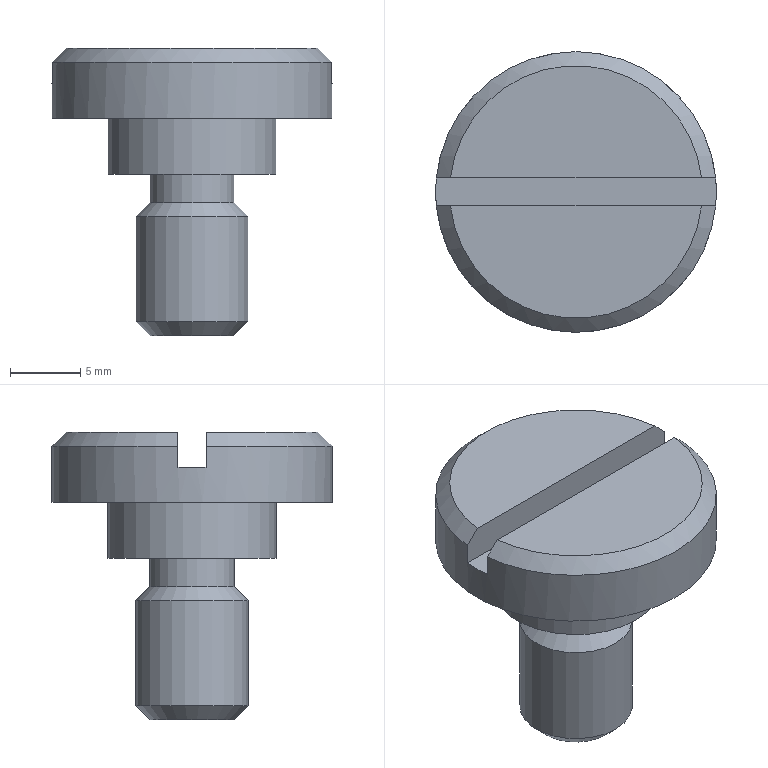Component | NX | DRILL_BUSHING_SCREW | 1 solid | 16 faces | box 20 x 20 x 20.5 mm | volume 2406 mm3 | plane 8 | cylinder 4 | cone 4 | commonest cylinder face diameters 8 x1 6 x1 12 x1 20 x1
STEP:
#1=CARTESIAN_POINT('',(0.,0.,0.));
#2=DIRECTION('',(0.,0.,1.));
#3=DIRECTION('',(1.,0.,0.));
#4=AXIS2_PLACEMENT_3D('',#1,#2,#3);
#5=CARTESIAN_POINT('',(-8.944,49.,-79.));
#6=VERTEX_POINT('',#5);
#7=CARTESIAN_POINT('',(8.944,49.,-79.));
#8=VERTEX_POINT('',#7);
#9=CARTESIAN_POINT('',(-13.1,49.,-79.));
#10=DIRECTION('',(1.,-0.,0.));
#11=VECTOR('',#10,1.);
#12=LINE('',#9,#11);
#13=CARTESIAN_POINT('',(-0.,50.,-79.));
#14=DIRECTION('',(0.,0.,1.));
#15=DIRECTION('',(0.,1.,0.));
#16=AXIS2_PLACEMENT_3D('',#13,#14,#15);
#17=PLANE('',#16);
#18=CARTESIAN_POINT('',(-1.,13.1));
#19=DIRECTION('',(-0.,-1.));
#20=VECTOR('',#19,1.);
#21=LINE('',#18,#20);
#22=(GEOMETRIC_REPRESENTATION_CONTEXT(2)PARAMETRIC_REPRESENTATION_CONTEXT()REPRESENTATION_CONTEXT('',''));
#23=DEFINITIONAL_REPRESENTATION('',(#21),#22);
#24=PCURVE('',#17,#23);
#25=CARTESIAN_POINT('',(-13.1,49.,-81.5));
#26=DIRECTION('',(-0.,-1.,0.));
#27=DIRECTION('',(1.,-0.,0.));
#28=AXIS2_PLACEMENT_3D('',#25,#26,#27);
#29=PLANE('',#28);
#30=CARTESIAN_POINT('',(0.,2.5));
#31=DIRECTION('',(1.,0.));
#32=VECTOR('',#31,1.);
#33=LINE('',#30,#32);
#34=(GEOMETRIC_REPRESENTATION_CONTEXT(2)PARAMETRIC_REPRESENTATION_CONTEXT()REPRESENTATION_CONTEXT('',''));
#35=DEFINITIONAL_REPRESENTATION('',(#33),#34);
#36=PCURVE('',#29,#35);
#37=SURFACE_CURVE('',#12,(#24,#36),.PCURVE_S1.);
#38=EDGE_CURVE('',#6,#8,#37,.T.);
#39=ORIENTED_EDGE('',*,*,#38,.F.);
#40=CARTESIAN_POINT('',(-0.,50.,-79.));
#41=DIRECTION('',(0.,0.,1.));
#42=DIRECTION('',(0.,1.,0.));
#43=AXIS2_PLACEMENT_3D('',#40,#41,#42);
#44=CIRCLE('',#43,9.);
#45=CARTESIAN_POINT('',(0.,0.));
#46=DIRECTION('',(1.,0.));
#47=AXIS2_PLACEMENT_2D('',#45,#46);
#48=CIRCLE('',#47,9.);
#49=(GEOMETRIC_REPRESENTATION_CONTEXT(2)PARAMETRIC_REPRESENTATION_CONTEXT()REPRESENTATION_CONTEXT('',''));
#50=DEFINITIONAL_REPRESENTATION('',(#48),#49);
#51=PCURVE('',#17,#50);
#52=CARTESIAN_POINT('',(-0.,50.,-79.));
#53=DIRECTION('',(0.,0.,-1.));
#54=DIRECTION('',(0.,-1.,0.));
#55=AXIS2_PLACEMENT_3D('',#52,#53,#54);
#56=CONICAL_SURFACE('',#55,9.,0.7854);
#57=CARTESIAN_POINT('',(3.142,0.));
#58=DIRECTION('',(-1.,0.));
#59=VECTOR('',#58,1.);
#60=LINE('',#57,#59);
#61=(GEOMETRIC_REPRESENTATION_CONTEXT(2)PARAMETRIC_REPRESENTATION_CONTEXT()REPRESENTATION_CONTEXT('',''));
#62=DEFINITIONAL_REPRESENTATION('',(#60),#61);
#63=PCURVE('',#56,#62);
#64=SURFACE_CURVE('',#44,(#51,#63),.PCURVE_S1.);
#65=EDGE_CURVE('',#6,#8,#64,.T.);
#66=ORIENTED_EDGE('',*,*,#65,.T.);
#67=EDGE_LOOP('',(#39,#66));
#68=FACE_BOUND('',#67,.T.);
#69=ADVANCED_FACE('',(#68),#17,.T.);
#70=CARTESIAN_POINT('',(-0.,54.,-98.5));
#71=VERTEX_POINT('',#70);
#72=CARTESIAN_POINT('',(-0.,50.,-98.5));
#73=DIRECTION('',(0.,0.,1.));
#74=DIRECTION('',(0.,1.,0.));
#75=AXIS2_PLACEMENT_3D('',#72,#73,#74);
#76=CIRCLE('',#75,4.);
#77=CARTESIAN_POINT('',(-0.,50.,-90.));
#78=DIRECTION('',(0.,0.,-1.));
#79=DIRECTION('',(0.,-1.,0.));
#80=AXIS2_PLACEMENT_3D('',#77,#78,#79);
#81=CYLINDRICAL_SURFACE('',#80,4.);
#82=CARTESIAN_POINT('',(9.425,8.5));
#83=DIRECTION('',(-1.,0.));
#84=VECTOR('',#83,1.);
#85=LINE('',#82,#84);
#86=(GEOMETRIC_REPRESENTATION_CONTEXT(2)PARAMETRIC_REPRESENTATION_CONTEXT()REPRESENTATION_CONTEXT('',''));
#87=DEFINITIONAL_REPRESENTATION('',(#85),#86);
#88=PCURVE('',#81,#87);
#89=CARTESIAN_POINT('',(-0.,50.,-98.5));
#90=DIRECTION('',(0.,0.,1.));
#91=DIRECTION('',(0.,1.,0.));
#92=AXIS2_PLACEMENT_3D('',#89,#90,#91);
#93=CONICAL_SURFACE('',#92,4.,0.7854);
#94=CARTESIAN_POINT('',(0.,0.));
#95=DIRECTION('',(1.,0.));
#96=VECTOR('',#95,1.);
#97=LINE('',#94,#96);
#98=(GEOMETRIC_REPRESENTATION_CONTEXT(2)PARAMETRIC_REPRESENTATION_CONTEXT()REPRESENTATION_CONTEXT('',''));
#99=DEFINITIONAL_REPRESENTATION('',(#97),#98);
#100=PCURVE('',#93,#99);
#101=SURFACE_CURVE('',#76,(#88,#100),.PCURVE_S1.);
#102=EDGE_CURVE('',#71,#71,#101,.T.);
#103=ORIENTED_EDGE('',*,*,#102,.T.);
#104=CARTESIAN_POINT('',(-0.,54.,-91.));
#105=VERTEX_POINT('',#104);
#106=CARTESIAN_POINT('',(-0.,54.,-91.));
#107=CARTESIAN_POINT('',(-0.,54.,-98.5));
#108=B_SPLINE_CURVE_WITH_KNOTS('',1,(#106,#107),.UNSPECIFIED.,.F.,.F.,(2,2),(1.,8.5),.PIECEWISE_BEZIER_KNOTS.);
#109=CARTESIAN_POINT('',(3.142,0.));
#110=DIRECTION('',(0.,1.));
#111=VECTOR('',#110,1.);
#112=LINE('',#109,#111);
#113=(GEOMETRIC_REPRESENTATION_CONTEXT(2)PARAMETRIC_REPRESENTATION_CONTEXT()REPRESENTATION_CONTEXT('',''));
#114=DEFINITIONAL_REPRESENTATION('',(#112),#113);
#115=PCURVE('',#81,#114);
#116=CARTESIAN_POINT('',(9.425,0.));
#117=DIRECTION('',(0.,1.));
#118=VECTOR('',#117,1.);
#119=LINE('',#116,#118);
#120=(GEOMETRIC_REPRESENTATION_CONTEXT(2)PARAMETRIC_REPRESENTATION_CONTEXT()REPRESENTATION_CONTEXT('',''));
#121=DEFINITIONAL_REPRESENTATION('',(#119),#120);
#122=PCURVE('',#81,#121);
#123=SEAM_CURVE('',#108,(#115,#122),.PCURVE_S1.);
#124=EDGE_CURVE('',#105,#71,#123,.T.);
#125=ORIENTED_EDGE('',*,*,#124,.F.);
#126=CARTESIAN_POINT('',(-0.,50.,-91.));
#127=DIRECTION('',(0.,0.,-1.));
#128=DIRECTION('',(0.,1.,0.));
#129=AXIS2_PLACEMENT_3D('',#126,#127,#128);
#130=CIRCLE('',#129,4.);
#131=CARTESIAN_POINT('',(3.142,1.));
#132=DIRECTION('',(1.,0.));
#133=VECTOR('',#132,1.);
#134=LINE('',#131,#133);
#135=(GEOMETRIC_REPRESENTATION_CONTEXT(2)PARAMETRIC_REPRESENTATION_CONTEXT()REPRESENTATION_CONTEXT('',''));
#136=DEFINITIONAL_REPRESENTATION('',(#134),#135);
#137=PCURVE('',#81,#136);
#138=CARTESIAN_POINT('',(-0.,50.,-90.));
#139=DIRECTION('',(0.,0.,-1.));
#140=DIRECTION('',(0.,-1.,0.));
#141=AXIS2_PLACEMENT_3D('',#138,#139,#140);
#142=CONICAL_SURFACE('',#141,3.,0.7854);
#143=CARTESIAN_POINT('',(3.142,1.));
#144=DIRECTION('',(1.,0.));
#145=VECTOR('',#144,1.);
#146=LINE('',#143,#145);
#147=(GEOMETRIC_REPRESENTATION_CONTEXT(2)PARAMETRIC_REPRESENTATION_CONTEXT()REPRESENTATION_CONTEXT('',''));
#148=DEFINITIONAL_REPRESENTATION('',(#146),#147);
#149=PCURVE('',#142,#148);
#150=SURFACE_CURVE('',#130,(#137,#149),.PCURVE_S1.);
#151=EDGE_CURVE('',#105,#105,#150,.T.);
#152=ORIENTED_EDGE('',*,*,#151,.T.);
#153=ORIENTED_EDGE('',*,*,#124,.T.);
#154=EDGE_LOOP('',(#103,#125,#152,#153));
#155=FACE_BOUND('',#154,.T.);
#156=ADVANCED_FACE('',(#155),#81,.T.);
#157=CARTESIAN_POINT('',(-0.,53.,-99.5));
#158=VERTEX_POINT('',#157);
#159=CARTESIAN_POINT('',(-0.,50.,-99.5));
#160=DIRECTION('',(0.,0.,-1.));
#161=DIRECTION('',(0.,1.,0.));
#162=AXIS2_PLACEMENT_3D('',#159,#160,#161);
#163=CIRCLE('',#162,3.);
#164=CARTESIAN_POINT('',(-0.,50.,-99.5));
#165=DIRECTION('',(0.,0.,1.));
#166=DIRECTION('',(0.,1.,0.));
#167=AXIS2_PLACEMENT_3D('',#164,#165,#166);
#168=PLANE('',#167);
#169=CARTESIAN_POINT('',(3.,0.));
#170=CARTESIAN_POINT('',(3.,-5.196));
#171=CARTESIAN_POINT('',(-1.5,-2.598));
#172=CARTESIAN_POINT('',(-6.,-0.));
#173=CARTESIAN_POINT('',(-1.5,2.598));
#174=CARTESIAN_POINT('',(3.,5.196));
#175=CARTESIAN_POINT('',(3.,0.));
#176=(BOUNDED_CURVE()B_SPLINE_CURVE(2,(#169,#170,#171,#172,#173,#174,#175),.UNSPECIFIED.,.T.,.F.)B_SPLINE_CURVE_WITH_KNOTS((1,2,2,2,2,1),(-2.094,0.,2.094,4.189,6.283,8.378),.UNSPECIFIED.)CURVE()GEOMETRIC_REPRESENTATION_ITEM()RATIONAL_B_SPLINE_CURVE((1.,0.5,1.,0.5,1.,0.5,1.))REPRESENTATION_ITEM(''));
#177=(GEOMETRIC_REPRESENTATION_CONTEXT(2)PARAMETRIC_REPRESENTATION_CONTEXT()REPRESENTATION_CONTEXT('',''));
#178=DEFINITIONAL_REPRESENTATION('',(#176),#177);
#179=PCURVE('',#168,#178);
#180=CARTESIAN_POINT('',(6.283,-1.));
#181=DIRECTION('',(-1.,0.));
#182=VECTOR('',#181,1.);
#183=LINE('',#180,#182);
#184=(GEOMETRIC_REPRESENTATION_CONTEXT(2)PARAMETRIC_REPRESENTATION_CONTEXT()REPRESENTATION_CONTEXT('',''));
#185=DEFINITIONAL_REPRESENTATION('',(#183),#184);
#186=PCURVE('',#93,#185);
#187=SURFACE_CURVE('',#163,(#179,#186),.PCURVE_S1.);
#188=EDGE_CURVE('',#158,#158,#187,.T.);
#189=ORIENTED_EDGE('',*,*,#188,.T.);
#190=EDGE_LOOP('',(#189));
#191=FACE_BOUND('',#190,.T.);
#192=ADVANCED_FACE('',(#191),#168,.F.);
#193=CARTESIAN_POINT('',(-0.,53.,-88.));
#194=VERTEX_POINT('',#193);
#195=CARTESIAN_POINT('',(-0.,50.,-88.));
#196=DIRECTION('',(0.,0.,1.));
#197=DIRECTION('',(0.,1.,0.));
#198=AXIS2_PLACEMENT_3D('',#195,#196,#197);
#199=CIRCLE('',#198,3.);
#200=CARTESIAN_POINT('',(-0.,50.,-88.));
#201=DIRECTION('',(0.,0.,-1.));
#202=DIRECTION('',(0.,-1.,0.));
#203=AXIS2_PLACEMENT_3D('',#200,#201,#202);
#204=CYLINDRICAL_SURFACE('',#203,3.);
#205=CARTESIAN_POINT('',(9.425,0.));
#206=DIRECTION('',(-1.,0.));
#207=VECTOR('',#206,1.);
#208=LINE('',#205,#207);
#209=(GEOMETRIC_REPRESENTATION_CONTEXT(2)PARAMETRIC_REPRESENTATION_CONTEXT()REPRESENTATION_CONTEXT('',''));
#210=DEFINITIONAL_REPRESENTATION('',(#208),#209);
#211=PCURVE('',#204,#210);
#212=CARTESIAN_POINT('',(-0.,50.,-88.));
#213=DIRECTION('',(0.,0.,1.));
#214=DIRECTION('',(0.,1.,0.));
#215=AXIS2_PLACEMENT_3D('',#212,#213,#214);
#216=PLANE('',#215);
#217=CARTESIAN_POINT('',(0.,0.));
#218=DIRECTION('',(1.,0.));
#219=AXIS2_PLACEMENT_2D('',#217,#218);
#220=CIRCLE('',#219,3.);
#221=(GEOMETRIC_REPRESENTATION_CONTEXT(2)PARAMETRIC_REPRESENTATION_CONTEXT()REPRESENTATION_CONTEXT('',''));
#222=DEFINITIONAL_REPRESENTATION('',(#220),#221);
#223=PCURVE('',#216,#222);
#224=SURFACE_CURVE('',#199,(#211,#223),.PCURVE_S1.);
#225=EDGE_CURVE('',#194,#194,#224,.T.);
#226=ORIENTED_EDGE('',*,*,#225,.F.);
#227=CARTESIAN_POINT('',(-0.,53.,-90.));
#228=VERTEX_POINT('',#227);
#229=CARTESIAN_POINT('',(-0.,53.,-88.));
#230=CARTESIAN_POINT('',(-0.,53.,-90.));
#231=B_SPLINE_CURVE_WITH_KNOTS('',1,(#229,#230),.UNSPECIFIED.,.F.,.F.,(2,2),(0.,2.),.PIECEWISE_BEZIER_KNOTS.);
#232=CARTESIAN_POINT('',(9.425,0.));
#233=DIRECTION('',(0.,1.));
#234=VECTOR('',#233,1.);
#235=LINE('',#232,#234);
#236=(GEOMETRIC_REPRESENTATION_CONTEXT(2)PARAMETRIC_REPRESENTATION_CONTEXT()REPRESENTATION_CONTEXT('',''));
#237=DEFINITIONAL_REPRESENTATION('',(#235),#236);
#238=PCURVE('',#204,#237);
#239=CARTESIAN_POINT('',(3.142,0.));
#240=DIRECTION('',(0.,1.));
#241=VECTOR('',#240,1.);
#242=LINE('',#239,#241);
#243=(GEOMETRIC_REPRESENTATION_CONTEXT(2)PARAMETRIC_REPRESENTATION_CONTEXT()REPRESENTATION_CONTEXT('',''));
#244=DEFINITIONAL_REPRESENTATION('',(#242),#243);
#245=PCURVE('',#204,#244);
#246=SEAM_CURVE('',#231,(#238,#245),.PCURVE_S1.);
#247=EDGE_CURVE('',#194,#228,#246,.T.);
#248=ORIENTED_EDGE('',*,*,#247,.T.);
#249=CARTESIAN_POINT('',(-0.,50.,-90.));
#250=DIRECTION('',(0.,0.,1.));
#251=DIRECTION('',(0.,1.,0.));
#252=AXIS2_PLACEMENT_3D('',#249,#250,#251);
#253=CIRCLE('',#252,3.);
#254=CARTESIAN_POINT('',(9.425,2.));
#255=DIRECTION('',(-1.,0.));
#256=VECTOR('',#255,1.);
#257=LINE('',#254,#256);
#258=(GEOMETRIC_REPRESENTATION_CONTEXT(2)PARAMETRIC_REPRESENTATION_CONTEXT()REPRESENTATION_CONTEXT('',''));
#259=DEFINITIONAL_REPRESENTATION('',(#257),#258);
#260=PCURVE('',#204,#259);
#261=CARTESIAN_POINT('',(9.425,0.));
#262=DIRECTION('',(-1.,0.));
#263=VECTOR('',#262,1.);
#264=LINE('',#261,#263);
#265=(GEOMETRIC_REPRESENTATION_CONTEXT(2)PARAMETRIC_REPRESENTATION_CONTEXT()REPRESENTATION_CONTEXT('',''));
#266=DEFINITIONAL_REPRESENTATION('',(#264),#265);
#267=PCURVE('',#142,#266);
#268=SURFACE_CURVE('',#253,(#260,#267),.PCURVE_S1.);
#269=EDGE_CURVE('',#228,#228,#268,.T.);
#270=ORIENTED_EDGE('',*,*,#269,.T.);
#271=ORIENTED_EDGE('',*,*,#247,.F.);
#272=EDGE_LOOP('',(#226,#248,#270,#271));
#273=FACE_BOUND('',#272,.T.);
#274=ADVANCED_FACE('',(#273),#204,.T.);
#275=CARTESIAN_POINT('',(-0.,56.,-84.));
#276=VERTEX_POINT('',#275);
#277=CARTESIAN_POINT('',(-0.,50.,-84.));
#278=DIRECTION('',(0.,0.,1.));
#279=DIRECTION('',(0.,1.,0.));
#280=AXIS2_PLACEMENT_3D('',#277,#278,#279);
#281=CIRCLE('',#280,6.);
#282=CARTESIAN_POINT('',(-0.,50.,-84.));
#283=DIRECTION('',(0.,0.,-1.));
#284=DIRECTION('',(0.,-1.,0.));
#285=AXIS2_PLACEMENT_3D('',#282,#283,#284);
#286=CYLINDRICAL_SURFACE('',#285,6.);
#287=CARTESIAN_POINT('',(9.425,0.));
#288=DIRECTION('',(-1.,0.));
#289=VECTOR('',#288,1.);
#290=LINE('',#287,#289);
#291=(GEOMETRIC_REPRESENTATION_CONTEXT(2)PARAMETRIC_REPRESENTATION_CONTEXT()REPRESENTATION_CONTEXT('',''));
#292=DEFINITIONAL_REPRESENTATION('',(#290),#291);
#293=PCURVE('',#286,#292);
#294=CARTESIAN_POINT('',(-0.,50.,-84.));
#295=DIRECTION('',(0.,0.,1.));
#296=DIRECTION('',(0.,1.,0.));
#297=AXIS2_PLACEMENT_3D('',#294,#295,#296);
#298=PLANE('',#297);
#299=CARTESIAN_POINT('',(0.,0.));
#300=DIRECTION('',(1.,0.));
#301=AXIS2_PLACEMENT_2D('',#299,#300);
#302=CIRCLE('',#301,6.);
#303=(GEOMETRIC_REPRESENTATION_CONTEXT(2)PARAMETRIC_REPRESENTATION_CONTEXT()REPRESENTATION_CONTEXT('',''));
#304=DEFINITIONAL_REPRESENTATION('',(#302),#303);
#305=PCURVE('',#298,#304);
#306=SURFACE_CURVE('',#281,(#293,#305),.PCURVE_S1.);
#307=EDGE_CURVE('',#276,#276,#306,.T.);
#308=ORIENTED_EDGE('',*,*,#307,.F.);
#309=CARTESIAN_POINT('',(-0.,56.,-88.));
#310=VERTEX_POINT('',#309);
#311=CARTESIAN_POINT('',(-0.,56.,-84.));
#312=CARTESIAN_POINT('',(-0.,56.,-88.));
#313=B_SPLINE_CURVE_WITH_KNOTS('',1,(#311,#312),.UNSPECIFIED.,.F.,.F.,(2,2),(0.,4.),.PIECEWISE_BEZIER_KNOTS.);
#314=CARTESIAN_POINT('',(9.425,0.));
#315=DIRECTION('',(0.,1.));
#316=VECTOR('',#315,1.);
#317=LINE('',#314,#316);
#318=(GEOMETRIC_REPRESENTATION_CONTEXT(2)PARAMETRIC_REPRESENTATION_CONTEXT()REPRESENTATION_CONTEXT('',''));
#319=DEFINITIONAL_REPRESENTATION('',(#317),#318);
#320=PCURVE('',#286,#319);
#321=CARTESIAN_POINT('',(3.142,0.));
#322=DIRECTION('',(0.,1.));
#323=VECTOR('',#322,1.);
#324=LINE('',#321,#323);
#325=(GEOMETRIC_REPRESENTATION_CONTEXT(2)PARAMETRIC_REPRESENTATION_CONTEXT()REPRESENTATION_CONTEXT('',''));
#326=DEFINITIONAL_REPRESENTATION('',(#324),#325);
#327=PCURVE('',#286,#326);
#328=SEAM_CURVE('',#313,(#320,#327),.PCURVE_S1.);
#329=EDGE_CURVE('',#276,#310,#328,.T.);
#330=ORIENTED_EDGE('',*,*,#329,.T.);
#331=CARTESIAN_POINT('',(-0.,50.,-88.));
#332=DIRECTION('',(0.,0.,1.));
#333=DIRECTION('',(0.,1.,0.));
#334=AXIS2_PLACEMENT_3D('',#331,#332,#333);
#335=CIRCLE('',#334,6.);
#336=CARTESIAN_POINT('',(9.425,4.));
#337=DIRECTION('',(-1.,0.));
#338=VECTOR('',#337,1.);
#339=LINE('',#336,#338);
#340=(GEOMETRIC_REPRESENTATION_CONTEXT(2)PARAMETRIC_REPRESENTATION_CONTEXT()REPRESENTATION_CONTEXT('',''));
#341=DEFINITIONAL_REPRESENTATION('',(#339),#340);
#342=PCURVE('',#286,#341);
#343=CARTESIAN_POINT('',(0.,0.));
#344=DIRECTION('',(1.,0.));
#345=AXIS2_PLACEMENT_2D('',#343,#344);
#346=CIRCLE('',#345,6.);
#347=(GEOMETRIC_REPRESENTATION_CONTEXT(2)PARAMETRIC_REPRESENTATION_CONTEXT()REPRESENTATION_CONTEXT('',''));
#348=DEFINITIONAL_REPRESENTATION('',(#346),#347);
#349=PCURVE('',#216,#348);
#350=SURFACE_CURVE('',#335,(#342,#349),.PCURVE_S1.);
#351=EDGE_CURVE('',#310,#310,#350,.T.);
#352=ORIENTED_EDGE('',*,*,#351,.T.);
#353=ORIENTED_EDGE('',*,*,#329,.F.);
#354=EDGE_LOOP('',(#308,#330,#352,#353));
#355=FACE_BOUND('',#354,.T.);
#356=ADVANCED_FACE('',(#355),#286,.T.);
#357=ORIENTED_EDGE('',*,*,#225,.T.);
#358=EDGE_LOOP('',(#357));
#359=FACE_BOUND('',#358,.T.);
#360=ORIENTED_EDGE('',*,*,#351,.F.);
#361=EDGE_LOOP('',(#360));
#362=FACE_BOUND('',#361,.T.);
#363=ADVANCED_FACE('',(#359,#362),#216,.F.);
#364=CARTESIAN_POINT('',(-9.95,51.,-81.5));
#365=VERTEX_POINT('',#364);
#366=CARTESIAN_POINT('',(-9.95,51.,-80.));
#367=VERTEX_POINT('',#366);
#368=CARTESIAN_POINT('',(-9.95,51.,-79.));
#369=DIRECTION('',(0.,0.,1.));
#370=VECTOR('',#369,1.);
#371=LINE('',#368,#370);
#372=CARTESIAN_POINT('',(-0.,50.,-79.));
#373=DIRECTION('',(0.,0.,-1.));
#374=DIRECTION('',(0.,-1.,0.));
#375=AXIS2_PLACEMENT_3D('',#372,#373,#374);
#376=CYLINDRICAL_SURFACE('',#375,10.);
#377=CARTESIAN_POINT('',(7.954,0.));
#378=DIRECTION('',(0.,-1.));
#379=VECTOR('',#378,1.);
#380=LINE('',#377,#379);
#381=(GEOMETRIC_REPRESENTATION_CONTEXT(2)PARAMETRIC_REPRESENTATION_CONTEXT()REPRESENTATION_CONTEXT('',''));
#382=DEFINITIONAL_REPRESENTATION('',(#380),#381);
#383=PCURVE('',#376,#382);
#384=CARTESIAN_POINT('',(11.5,51.,-81.5));
#385=DIRECTION('',(-0.,1.,0.));
#386=DIRECTION('',(-1.,-0.,0.));
#387=AXIS2_PLACEMENT_3D('',#384,#385,#386);
#388=PLANE('',#387);
#389=CARTESIAN_POINT('',(21.45,2.5));
#390=DIRECTION('',(0.,1.));
#391=VECTOR('',#390,1.);
#392=LINE('',#389,#391);
#393=(GEOMETRIC_REPRESENTATION_CONTEXT(2)PARAMETRIC_REPRESENTATION_CONTEXT()REPRESENTATION_CONTEXT('',''));
#394=DEFINITIONAL_REPRESENTATION('',(#392),#393);
#395=PCURVE('',#388,#394);
#396=SURFACE_CURVE('',#371,(#383,#395),.PCURVE_S1.);
#397=EDGE_CURVE('',#365,#367,#396,.T.);
#398=ORIENTED_EDGE('',*,*,#397,.T.);
#399=CARTESIAN_POINT('',(9.95,51.,-80.));
#400=VERTEX_POINT('',#399);
#401=CARTESIAN_POINT('',(-0.,50.,-80.));
#402=DIRECTION('',(0.,0.,-1.));
#403=DIRECTION('',(0.,1.,0.));
#404=AXIS2_PLACEMENT_3D('',#401,#402,#403);
#405=CIRCLE('',#404,10.);
#406=CARTESIAN_POINT('',(3.142,1.));
#407=DIRECTION('',(1.,0.));
#408=VECTOR('',#407,1.);
#409=LINE('',#406,#408);
#410=(GEOMETRIC_REPRESENTATION_CONTEXT(2)PARAMETRIC_REPRESENTATION_CONTEXT()REPRESENTATION_CONTEXT('',''));
#411=DEFINITIONAL_REPRESENTATION('',(#409),#410);
#412=PCURVE('',#376,#411);
#413=CARTESIAN_POINT('',(-0.,50.,-79.));
#414=DIRECTION('',(0.,0.,-1.));
#415=DIRECTION('',(0.,-1.,0.));
#416=AXIS2_PLACEMENT_3D('',#413,#414,#415);
#417=CONICAL_SURFACE('',#416,9.,0.7854);
#418=CARTESIAN_POINT('',(-3.142,1.));
#419=DIRECTION('',(1.,0.));
#420=VECTOR('',#419,1.);
#421=LINE('',#418,#420);
#422=(GEOMETRIC_REPRESENTATION_CONTEXT(2)PARAMETRIC_REPRESENTATION_CONTEXT()REPRESENTATION_CONTEXT('',''));
#423=DEFINITIONAL_REPRESENTATION('',(#421),#422);
#424=PCURVE('',#417,#423);
#425=SURFACE_CURVE('',#405,(#412,#424),.PCURVE_S1.);
#426=EDGE_CURVE('',#367,#400,#425,.T.);
#427=ORIENTED_EDGE('',*,*,#426,.T.);
#428=CARTESIAN_POINT('',(9.95,51.,-81.5));
#429=VERTEX_POINT('',#428);
#430=CARTESIAN_POINT('',(9.95,51.,-79.));
#431=DIRECTION('',(0.,0.,-1.));
#432=VECTOR('',#431,1.);
#433=LINE('',#430,#432);
#434=CARTESIAN_POINT('',(10.895,0.));
#435=DIRECTION('',(0.,1.));
#436=VECTOR('',#435,1.);
#437=LINE('',#434,#436);
#438=(GEOMETRIC_REPRESENTATION_CONTEXT(2)PARAMETRIC_REPRESENTATION_CONTEXT()REPRESENTATION_CONTEXT('',''));
#439=DEFINITIONAL_REPRESENTATION('',(#437),#438);
#440=PCURVE('',#376,#439);
#441=CARTESIAN_POINT('',(1.55,2.5));
#442=DIRECTION('',(0.,-1.));
#443=VECTOR('',#442,1.);
#444=LINE('',#441,#443);
#445=(GEOMETRIC_REPRESENTATION_CONTEXT(2)PARAMETRIC_REPRESENTATION_CONTEXT()REPRESENTATION_CONTEXT('',''));
#446=DEFINITIONAL_REPRESENTATION('',(#444),#445);
#447=PCURVE('',#388,#446);
#448=SURFACE_CURVE('',#433,(#440,#447),.PCURVE_S1.);
#449=EDGE_CURVE('',#400,#429,#448,.T.);
#450=ORIENTED_EDGE('',*,*,#449,.T.);
#451=CARTESIAN_POINT('',(9.95,49.,-81.5));
#452=VERTEX_POINT('',#451);
#453=CARTESIAN_POINT('',(-0.,50.,-81.5));
#454=DIRECTION('',(0.,0.,1.));
#455=DIRECTION('',(0.,1.,0.));
#456=AXIS2_PLACEMENT_3D('',#453,#454,#455);
#457=CIRCLE('',#456,10.);
#458=CARTESIAN_POINT('',(15.708,2.5));
#459=DIRECTION('',(-1.,0.));
#460=VECTOR('',#459,1.);
#461=LINE('',#458,#460);
#462=(GEOMETRIC_REPRESENTATION_CONTEXT(2)PARAMETRIC_REPRESENTATION_CONTEXT()REPRESENTATION_CONTEXT('',''));
#463=DEFINITIONAL_REPRESENTATION('',(#461),#462);
#464=PCURVE('',#376,#463);
#465=CARTESIAN_POINT('',(-0.,50.,-81.5));
#466=DIRECTION('',(0.,0.,1.));
#467=DIRECTION('',(0.,1.,0.));
#468=AXIS2_PLACEMENT_3D('',#465,#466,#467);
#469=PLANE('',#468);
#470=CARTESIAN_POINT('',(0.,0.));
#471=DIRECTION('',(1.,0.));
#472=AXIS2_PLACEMENT_2D('',#470,#471);
#473=CIRCLE('',#472,10.);
#474=(GEOMETRIC_REPRESENTATION_CONTEXT(2)PARAMETRIC_REPRESENTATION_CONTEXT()REPRESENTATION_CONTEXT('',''));
#475=DEFINITIONAL_REPRESENTATION('',(#473),#474);
#476=PCURVE('',#469,#475);
#477=SURFACE_CURVE('',#457,(#464,#476),.PCURVE_S1.);
#478=EDGE_CURVE('',#452,#429,#477,.T.);
#479=ORIENTED_EDGE('',*,*,#478,.F.);
#480=CARTESIAN_POINT('',(9.95,49.,-84.));
#481=VERTEX_POINT('',#480);
#482=CARTESIAN_POINT('',(9.95,49.,-81.5));
#483=CARTESIAN_POINT('',(9.95,49.,-84.));
#484=B_SPLINE_CURVE_WITH_KNOTS('',1,(#482,#483),.UNSPECIFIED.,.F.,.F.,(2,2),(2.5,5.),.PIECEWISE_BEZIER_KNOTS.);
#485=CARTESIAN_POINT('',(11.096,0.));
#486=DIRECTION('',(0.,1.));
#487=VECTOR('',#486,1.);
#488=LINE('',#485,#487);
#489=(GEOMETRIC_REPRESENTATION_CONTEXT(2)PARAMETRIC_REPRESENTATION_CONTEXT()REPRESENTATION_CONTEXT('',''));
#490=DEFINITIONAL_REPRESENTATION('',(#488),#489);
#491=PCURVE('',#376,#490);
#492=CARTESIAN_POINT('',(4.813,0.));
#493=DIRECTION('',(0.,1.));
#494=VECTOR('',#493,1.);
#495=LINE('',#492,#494);
#496=(GEOMETRIC_REPRESENTATION_CONTEXT(2)PARAMETRIC_REPRESENTATION_CONTEXT()REPRESENTATION_CONTEXT('',''));
#497=DEFINITIONAL_REPRESENTATION('',(#495),#496);
#498=PCURVE('',#376,#497);
#499=SEAM_CURVE('',#484,(#491,#498),.PCURVE_S1.);
#500=EDGE_CURVE('',#452,#481,#499,.T.);
#501=ORIENTED_EDGE('',*,*,#500,.T.);
#502=CARTESIAN_POINT('',(-0.,60.,-84.));
#503=VERTEX_POINT('',#502);
#504=CARTESIAN_POINT('',(-0.,50.,-84.));
#505=DIRECTION('',(0.,0.,1.));
#506=DIRECTION('',(0.,1.,0.));
#507=AXIS2_PLACEMENT_3D('',#504,#505,#506);
#508=CIRCLE('',#507,10.);
#509=CARTESIAN_POINT('',(15.708,5.));
#510=DIRECTION('',(-1.,0.));
#511=VECTOR('',#510,1.);
#512=LINE('',#509,#511);
#513=(GEOMETRIC_REPRESENTATION_CONTEXT(2)PARAMETRIC_REPRESENTATION_CONTEXT()REPRESENTATION_CONTEXT('',''));
#514=DEFINITIONAL_REPRESENTATION('',(#512),#513);
#515=PCURVE('',#376,#514);
#516=CARTESIAN_POINT('',(0.,0.));
#517=DIRECTION('',(1.,0.));
#518=AXIS2_PLACEMENT_2D('',#516,#517);
#519=CIRCLE('',#518,10.);
#520=(GEOMETRIC_REPRESENTATION_CONTEXT(2)PARAMETRIC_REPRESENTATION_CONTEXT()REPRESENTATION_CONTEXT('',''));
#521=DEFINITIONAL_REPRESENTATION('',(#519),#520);
#522=PCURVE('',#298,#521);
#523=SURFACE_CURVE('',#508,(#515,#522),.PCURVE_S1.);
#524=EDGE_CURVE('',#481,#503,#523,.T.);
#525=ORIENTED_EDGE('',*,*,#524,.T.);
#526=CARTESIAN_POINT('',(-0.,50.,-84.));
#527=DIRECTION('',(0.,0.,1.));
#528=DIRECTION('',(0.,1.,0.));
#529=AXIS2_PLACEMENT_3D('',#526,#527,#528);
#530=CIRCLE('',#529,10.);
#531=CARTESIAN_POINT('',(9.425,5.));
#532=DIRECTION('',(-1.,0.));
#533=VECTOR('',#532,1.);
#534=LINE('',#531,#533);
#535=(GEOMETRIC_REPRESENTATION_CONTEXT(2)PARAMETRIC_REPRESENTATION_CONTEXT()REPRESENTATION_CONTEXT('',''));
#536=DEFINITIONAL_REPRESENTATION('',(#534),#535);
#537=PCURVE('',#376,#536);
#538=CARTESIAN_POINT('',(0.,0.));
#539=DIRECTION('',(1.,0.));
#540=AXIS2_PLACEMENT_2D('',#538,#539);
#541=CIRCLE('',#540,10.);
#542=(GEOMETRIC_REPRESENTATION_CONTEXT(2)PARAMETRIC_REPRESENTATION_CONTEXT()REPRESENTATION_CONTEXT('',''));
#543=DEFINITIONAL_REPRESENTATION('',(#541),#542);
#544=PCURVE('',#298,#543);
#545=SURFACE_CURVE('',#530,(#537,#544),.PCURVE_S1.);
#546=EDGE_CURVE('',#503,#481,#545,.T.);
#547=ORIENTED_EDGE('',*,*,#546,.T.);
#548=ORIENTED_EDGE('',*,*,#500,.F.);
#549=CARTESIAN_POINT('',(9.95,49.,-80.));
#550=VERTEX_POINT('',#549);
#551=CARTESIAN_POINT('',(9.95,49.,-79.));
#552=DIRECTION('',(0.,0.,1.));
#553=VECTOR('',#552,1.);
#554=LINE('',#551,#553);
#555=CARTESIAN_POINT('',(4.813,0.));
#556=DIRECTION('',(0.,-1.));
#557=VECTOR('',#556,1.);
#558=LINE('',#555,#557);
#559=(GEOMETRIC_REPRESENTATION_CONTEXT(2)PARAMETRIC_REPRESENTATION_CONTEXT()REPRESENTATION_CONTEXT('',''));
#560=DEFINITIONAL_REPRESENTATION('',(#558),#559);
#561=PCURVE('',#376,#560);
#562=CARTESIAN_POINT('',(23.05,2.5));
#563=DIRECTION('',(0.,1.));
#564=VECTOR('',#563,1.);
#565=LINE('',#562,#564);
#566=(GEOMETRIC_REPRESENTATION_CONTEXT(2)PARAMETRIC_REPRESENTATION_CONTEXT()REPRESENTATION_CONTEXT('',''));
#567=DEFINITIONAL_REPRESENTATION('',(#565),#566);
#568=PCURVE('',#29,#567);
#569=SURFACE_CURVE('',#554,(#561,#568),.PCURVE_S1.);
#570=EDGE_CURVE('',#452,#550,#569,.T.);
#571=ORIENTED_EDGE('',*,*,#570,.T.);
#572=CARTESIAN_POINT('',(-9.95,49.,-80.));
#573=VERTEX_POINT('',#572);
#574=CARTESIAN_POINT('',(-0.,50.,-80.));
#575=DIRECTION('',(0.,0.,-1.));
#576=DIRECTION('',(0.,1.,0.));
#577=AXIS2_PLACEMENT_3D('',#574,#575,#576);
#578=CIRCLE('',#577,10.);
#579=CARTESIAN_POINT('',(3.142,1.));
#580=DIRECTION('',(1.,0.));
#581=VECTOR('',#580,1.);
#582=LINE('',#579,#581);
#583=(GEOMETRIC_REPRESENTATION_CONTEXT(2)PARAMETRIC_REPRESENTATION_CONTEXT()REPRESENTATION_CONTEXT('',''));
#584=DEFINITIONAL_REPRESENTATION('',(#582),#583);
#585=PCURVE('',#376,#584);
#586=CARTESIAN_POINT('',(-3.142,1.));
#587=DIRECTION('',(1.,0.));
#588=VECTOR('',#587,1.);
#589=LINE('',#586,#588);
#590=(GEOMETRIC_REPRESENTATION_CONTEXT(2)PARAMETRIC_REPRESENTATION_CONTEXT()REPRESENTATION_CONTEXT('',''));
#591=DEFINITIONAL_REPRESENTATION('',(#589),#590);
#592=PCURVE('',#56,#591);
#593=SURFACE_CURVE('',#578,(#585,#592),.PCURVE_S1.);
#594=EDGE_CURVE('',#550,#573,#593,.T.);
#595=ORIENTED_EDGE('',*,*,#594,.T.);
#596=CARTESIAN_POINT('',(-9.95,49.,-81.5));
#597=VERTEX_POINT('',#596);
#598=CARTESIAN_POINT('',(-9.95,49.,-79.));
#599=DIRECTION('',(0.,0.,-1.));
#600=VECTOR('',#599,1.);
#601=LINE('',#598,#600);
#602=CARTESIAN_POINT('',(7.754,0.));
#603=DIRECTION('',(0.,1.));
#604=VECTOR('',#603,1.);
#605=LINE('',#602,#604);
#606=(GEOMETRIC_REPRESENTATION_CONTEXT(2)PARAMETRIC_REPRESENTATION_CONTEXT()REPRESENTATION_CONTEXT('',''));
#607=DEFINITIONAL_REPRESENTATION('',(#605),#606);
#608=PCURVE('',#376,#607);
#609=CARTESIAN_POINT('',(3.15,2.5));
#610=DIRECTION('',(0.,-1.));
#611=VECTOR('',#610,1.);
#612=LINE('',#609,#611);
#613=(GEOMETRIC_REPRESENTATION_CONTEXT(2)PARAMETRIC_REPRESENTATION_CONTEXT()REPRESENTATION_CONTEXT('',''));
#614=DEFINITIONAL_REPRESENTATION('',(#612),#613);
#615=PCURVE('',#29,#614);
#616=SURFACE_CURVE('',#601,(#608,#615),.PCURVE_S1.);
#617=EDGE_CURVE('',#573,#597,#616,.T.);
#618=ORIENTED_EDGE('',*,*,#617,.T.);
#619=CARTESIAN_POINT('',(-0.,50.,-81.5));
#620=DIRECTION('',(0.,0.,1.));
#621=DIRECTION('',(0.,1.,0.));
#622=AXIS2_PLACEMENT_3D('',#619,#620,#621);
#623=CIRCLE('',#622,10.);
#624=CARTESIAN_POINT('',(9.425,2.5));
#625=DIRECTION('',(-1.,0.));
#626=VECTOR('',#625,1.);
#627=LINE('',#624,#626);
#628=(GEOMETRIC_REPRESENTATION_CONTEXT(2)PARAMETRIC_REPRESENTATION_CONTEXT()REPRESENTATION_CONTEXT('',''));
#629=DEFINITIONAL_REPRESENTATION('',(#627),#628);
#630=PCURVE('',#376,#629);
#631=CARTESIAN_POINT('',(0.,0.));
#632=DIRECTION('',(1.,0.));
#633=AXIS2_PLACEMENT_2D('',#631,#632);
#634=CIRCLE('',#633,10.);
#635=(GEOMETRIC_REPRESENTATION_CONTEXT(2)PARAMETRIC_REPRESENTATION_CONTEXT()REPRESENTATION_CONTEXT('',''));
#636=DEFINITIONAL_REPRESENTATION('',(#634),#635);
#637=PCURVE('',#469,#636);
#638=SURFACE_CURVE('',#623,(#630,#637),.PCURVE_S1.);
#639=EDGE_CURVE('',#365,#597,#638,.T.);
#640=ORIENTED_EDGE('',*,*,#639,.F.);
#641=EDGE_LOOP('',(#398,#427,#450,#479,#501,#525,#547,#548,#571,#595,#618,#640));
#642=FACE_BOUND('',#641,.T.);
#643=ADVANCED_FACE('',(#642),#376,.T.);
#644=CARTESIAN_POINT('',(8.944,51.,-79.));
#645=VERTEX_POINT('',#644);
#646=CARTESIAN_POINT('',(-8.944,51.,-79.));
#647=VERTEX_POINT('',#646);
#648=CARTESIAN_POINT('',(11.5,51.,-79.));
#649=DIRECTION('',(-1.,-0.,0.));
#650=VECTOR('',#649,1.);
#651=LINE('',#648,#650);
#652=CARTESIAN_POINT('',(-0.,50.,-79.));
#653=DIRECTION('',(0.,0.,1.));
#654=DIRECTION('',(0.,1.,0.));
#655=AXIS2_PLACEMENT_3D('',#652,#653,#654);
#656=PLANE('',#655);
#657=CARTESIAN_POINT('',(1.,-11.5));
#658=DIRECTION('',(-0.,1.));
#659=VECTOR('',#658,1.);
#660=LINE('',#657,#659);
#661=(GEOMETRIC_REPRESENTATION_CONTEXT(2)PARAMETRIC_REPRESENTATION_CONTEXT()REPRESENTATION_CONTEXT('',''));
#662=DEFINITIONAL_REPRESENTATION('',(#660),#661);
#663=PCURVE('',#656,#662);
#664=CARTESIAN_POINT('',(0.,2.5));
#665=DIRECTION('',(1.,0.));
#666=VECTOR('',#665,1.);
#667=LINE('',#664,#666);
#668=(GEOMETRIC_REPRESENTATION_CONTEXT(2)PARAMETRIC_REPRESENTATION_CONTEXT()REPRESENTATION_CONTEXT('',''));
#669=DEFINITIONAL_REPRESENTATION('',(#667),#668);
#670=PCURVE('',#388,#669);
#671=SURFACE_CURVE('',#651,(#663,#670),.PCURVE_S1.);
#672=EDGE_CURVE('',#645,#647,#671,.T.);
#673=ORIENTED_EDGE('',*,*,#672,.F.);
#674=CARTESIAN_POINT('',(-0.,50.,-79.));
#675=DIRECTION('',(0.,0.,1.));
#676=DIRECTION('',(0.,1.,0.));
#677=AXIS2_PLACEMENT_3D('',#674,#675,#676);
#678=CIRCLE('',#677,9.);
#679=CARTESIAN_POINT('',(0.,0.));
#680=DIRECTION('',(1.,0.));
#681=AXIS2_PLACEMENT_2D('',#679,#680);
#682=CIRCLE('',#681,9.);
#683=(GEOMETRIC_REPRESENTATION_CONTEXT(2)PARAMETRIC_REPRESENTATION_CONTEXT()REPRESENTATION_CONTEXT('',''));
#684=DEFINITIONAL_REPRESENTATION('',(#682),#683);
#685=PCURVE('',#656,#684);
#686=CARTESIAN_POINT('',(9.425,0.));
#687=DIRECTION('',(-1.,0.));
#688=VECTOR('',#687,1.);
#689=LINE('',#686,#688);
#690=(GEOMETRIC_REPRESENTATION_CONTEXT(2)PARAMETRIC_REPRESENTATION_CONTEXT()REPRESENTATION_CONTEXT('',''));
#691=DEFINITIONAL_REPRESENTATION('',(#689),#690);
#692=PCURVE('',#417,#691);
#693=SURFACE_CURVE('',#678,(#685,#692),.PCURVE_S1.);
#694=EDGE_CURVE('',#645,#647,#693,.T.);
#695=ORIENTED_EDGE('',*,*,#694,.T.);
#696=EDGE_LOOP('',(#673,#695));
#697=FACE_BOUND('',#696,.T.);
#698=ADVANCED_FACE('',(#697),#656,.T.);
#699=ORIENTED_EDGE('',*,*,#307,.T.);
#700=EDGE_LOOP('',(#699));
#701=FACE_BOUND('',#700,.T.);
#702=ORIENTED_EDGE('',*,*,#546,.F.);
#703=ORIENTED_EDGE('',*,*,#524,.F.);
#704=EDGE_LOOP('',(#702,#703));
#705=FACE_BOUND('',#704,.T.);
#706=ADVANCED_FACE('',(#701,#705),#298,.F.);
#707=ORIENTED_EDGE('',*,*,#639,.T.);
#708=CARTESIAN_POINT('',(-13.1,49.,-81.5));
#709=DIRECTION('',(-1.,0.,0.));
#710=VECTOR('',#709,1.);
#711=LINE('',#708,#710);
#712=CARTESIAN_POINT('',(-1.,13.1));
#713=DIRECTION('',(0.,1.));
#714=VECTOR('',#713,1.);
#715=LINE('',#712,#714);
#716=(GEOMETRIC_REPRESENTATION_CONTEXT(2)PARAMETRIC_REPRESENTATION_CONTEXT()REPRESENTATION_CONTEXT('',''));
#717=DEFINITIONAL_REPRESENTATION('',(#715),#716);
#718=PCURVE('',#469,#717);
#719=CARTESIAN_POINT('',(0.,0.));
#720=DIRECTION('',(-1.,0.));
#721=VECTOR('',#720,1.);
#722=LINE('',#719,#721);
#723=(GEOMETRIC_REPRESENTATION_CONTEXT(2)PARAMETRIC_REPRESENTATION_CONTEXT()REPRESENTATION_CONTEXT('',''));
#724=DEFINITIONAL_REPRESENTATION('',(#722),#723);
#725=PCURVE('',#29,#724);
#726=SURFACE_CURVE('',#711,(#718,#725),.PCURVE_S1.);
#727=EDGE_CURVE('',#452,#597,#726,.T.);
#728=ORIENTED_EDGE('',*,*,#727,.F.);
#729=ORIENTED_EDGE('',*,*,#478,.T.);
#730=CARTESIAN_POINT('',(11.5,51.,-81.5));
#731=DIRECTION('',(1.,0.,0.));
#732=VECTOR('',#731,1.);
#733=LINE('',#730,#732);
#734=CARTESIAN_POINT('',(1.,-11.5));
#735=DIRECTION('',(0.,-1.));
#736=VECTOR('',#735,1.);
#737=LINE('',#734,#736);
#738=(GEOMETRIC_REPRESENTATION_CONTEXT(2)PARAMETRIC_REPRESENTATION_CONTEXT()REPRESENTATION_CONTEXT('',''));
#739=DEFINITIONAL_REPRESENTATION('',(#737),#738);
#740=PCURVE('',#469,#739);
#741=CARTESIAN_POINT('',(0.,0.));
#742=DIRECTION('',(-1.,0.));
#743=VECTOR('',#742,1.);
#744=LINE('',#741,#743);
#745=(GEOMETRIC_REPRESENTATION_CONTEXT(2)PARAMETRIC_REPRESENTATION_CONTEXT()REPRESENTATION_CONTEXT('',''));
#746=DEFINITIONAL_REPRESENTATION('',(#744),#745);
#747=PCURVE('',#388,#746);
#748=SURFACE_CURVE('',#733,(#740,#747),.PCURVE_S1.);
#749=EDGE_CURVE('',#365,#429,#748,.T.);
#750=ORIENTED_EDGE('',*,*,#749,.F.);
#751=EDGE_LOOP('',(#707,#728,#729,#750));
#752=FACE_BOUND('',#751,.T.);
#753=ADVANCED_FACE('',(#752),#469,.T.);
#754=ORIENTED_EDGE('',*,*,#38,.T.);
#755=CARTESIAN_POINT('',(8.944,49.,-79.));
#756=CARTESIAN_POINT('',(9.28,49.,-79.333));
#757=CARTESIAN_POINT('',(9.615,49.,-79.667));
#758=CARTESIAN_POINT('',(9.95,49.,-80.));
#759=B_SPLINE_CURVE_WITH_KNOTS('',3,(#755,#756,#757,#758),.UNSPECIFIED.,.F.,.F.,(4,4),(0.,1.),.PIECEWISE_BEZIER_KNOTS.);
#760=CARTESIAN_POINT('',(22.044,2.5));
#761=CARTESIAN_POINT('',(22.38,2.167));
#762=CARTESIAN_POINT('',(22.715,1.833));
#763=CARTESIAN_POINT('',(23.05,1.5));
#764=B_SPLINE_CURVE_WITH_KNOTS('',3,(#760,#761,#762,#763),.UNSPECIFIED.,.F.,.F.,(4,4),(0.,1.),.PIECEWISE_BEZIER_KNOTS.);
#765=(GEOMETRIC_REPRESENTATION_CONTEXT(2)PARAMETRIC_REPRESENTATION_CONTEXT()REPRESENTATION_CONTEXT('',''));
#766=DEFINITIONAL_REPRESENTATION('',(#764),#765);
#767=PCURVE('',#29,#766);
#768=CARTESIAN_POINT('',(-1.459,0.));
#769=CARTESIAN_POINT('',(-1.471,1.));
#770=B_SPLINE_CURVE_WITH_KNOTS('',1,(#768,#769),.UNSPECIFIED.,.F.,.F.,(2,2),(0.,1.),.PIECEWISE_BEZIER_KNOTS.);
#771=(GEOMETRIC_REPRESENTATION_CONTEXT(2)PARAMETRIC_REPRESENTATION_CONTEXT()REPRESENTATION_CONTEXT('',''));
#772=DEFINITIONAL_REPRESENTATION('',(#770),#771);
#773=PCURVE('',#56,#772);
#774=SURFACE_CURVE('',#759,(#767,#773),.PCURVE_S1.);
#775=EDGE_CURVE('',#8,#550,#774,.T.);
#776=ORIENTED_EDGE('',*,*,#775,.T.);
#777=ORIENTED_EDGE('',*,*,#570,.F.);
#778=ORIENTED_EDGE('',*,*,#727,.T.);
#779=ORIENTED_EDGE('',*,*,#617,.F.);
#780=CARTESIAN_POINT('',(-9.95,49.,-80.));
#781=CARTESIAN_POINT('',(-9.615,49.,-79.667));
#782=CARTESIAN_POINT('',(-9.28,49.,-79.333));
#783=CARTESIAN_POINT('',(-8.944,49.,-79.));
#784=B_SPLINE_CURVE_WITH_KNOTS('',3,(#780,#781,#782,#783),.UNSPECIFIED.,.F.,.F.,(4,4),(0.,1.),.PIECEWISE_BEZIER_KNOTS.);
#785=CARTESIAN_POINT('',(3.15,1.5));
#786=CARTESIAN_POINT('',(3.485,1.833));
#787=CARTESIAN_POINT('',(3.82,2.167));
#788=CARTESIAN_POINT('',(4.156,2.5));
#789=B_SPLINE_CURVE_WITH_KNOTS('',3,(#785,#786,#787,#788),.UNSPECIFIED.,.F.,.F.,(4,4),(0.,1.),.PIECEWISE_BEZIER_KNOTS.);
#790=(GEOMETRIC_REPRESENTATION_CONTEXT(2)PARAMETRIC_REPRESENTATION_CONTEXT()REPRESENTATION_CONTEXT('',''));
#791=DEFINITIONAL_REPRESENTATION('',(#789),#790);
#792=PCURVE('',#29,#791);
#793=CARTESIAN_POINT('',(1.471,1.));
#794=CARTESIAN_POINT('',(1.459,0.));
#795=B_SPLINE_CURVE_WITH_KNOTS('',1,(#793,#794),.UNSPECIFIED.,.F.,.F.,(2,2),(0.,1.),.PIECEWISE_BEZIER_KNOTS.);
#796=(GEOMETRIC_REPRESENTATION_CONTEXT(2)PARAMETRIC_REPRESENTATION_CONTEXT()REPRESENTATION_CONTEXT('',''));
#797=DEFINITIONAL_REPRESENTATION('',(#795),#796);
#798=PCURVE('',#56,#797);
#799=SURFACE_CURVE('',#784,(#792,#798),.PCURVE_S1.);
#800=EDGE_CURVE('',#573,#6,#799,.T.);
#801=ORIENTED_EDGE('',*,*,#800,.T.);
#802=EDGE_LOOP('',(#754,#776,#777,#778,#779,#801));
#803=FACE_BOUND('',#802,.T.);
#804=ADVANCED_FACE('',(#803),#29,.F.);
#805=ORIENTED_EDGE('',*,*,#672,.T.);
#806=CARTESIAN_POINT('',(-8.944,51.,-79.));
#807=CARTESIAN_POINT('',(-9.28,51.,-79.333));
#808=CARTESIAN_POINT('',(-9.615,51.,-79.667));
#809=CARTESIAN_POINT('',(-9.95,51.,-80.));
#810=B_SPLINE_CURVE_WITH_KNOTS('',3,(#806,#807,#808,#809),.UNSPECIFIED.,.F.,.F.,(4,4),(0.,1.),.PIECEWISE_BEZIER_KNOTS.);
#811=CARTESIAN_POINT('',(20.444,2.5));
#812=CARTESIAN_POINT('',(20.78,2.167));
#813=CARTESIAN_POINT('',(21.115,1.833));
#814=CARTESIAN_POINT('',(21.45,1.5));
#815=B_SPLINE_CURVE_WITH_KNOTS('',3,(#811,#812,#813,#814),.UNSPECIFIED.,.F.,.F.,(4,4),(0.,1.),.PIECEWISE_BEZIER_KNOTS.);
#816=(GEOMETRIC_REPRESENTATION_CONTEXT(2)PARAMETRIC_REPRESENTATION_CONTEXT()REPRESENTATION_CONTEXT('',''));
#817=DEFINITIONAL_REPRESENTATION('',(#815),#816);
#818=PCURVE('',#388,#817);
#819=CARTESIAN_POINT('',(1.682,0.));
#820=CARTESIAN_POINT('',(1.671,1.));
#821=B_SPLINE_CURVE_WITH_KNOTS('',1,(#819,#820),.UNSPECIFIED.,.F.,.F.,(2,2),(0.,1.),.PIECEWISE_BEZIER_KNOTS.);
#822=(GEOMETRIC_REPRESENTATION_CONTEXT(2)PARAMETRIC_REPRESENTATION_CONTEXT()REPRESENTATION_CONTEXT('',''));
#823=DEFINITIONAL_REPRESENTATION('',(#821),#822);
#824=PCURVE('',#417,#823);
#825=SURFACE_CURVE('',#810,(#818,#824),.PCURVE_S1.);
#826=EDGE_CURVE('',#647,#367,#825,.T.);
#827=ORIENTED_EDGE('',*,*,#826,.T.);
#828=ORIENTED_EDGE('',*,*,#397,.F.);
#829=ORIENTED_EDGE('',*,*,#749,.T.);
#830=ORIENTED_EDGE('',*,*,#449,.F.);
#831=CARTESIAN_POINT('',(9.95,51.,-80.));
#832=CARTESIAN_POINT('',(9.615,51.,-79.667));
#833=CARTESIAN_POINT('',(9.28,51.,-79.333));
#834=CARTESIAN_POINT('',(8.944,51.,-79.));
#835=B_SPLINE_CURVE_WITH_KNOTS('',3,(#831,#832,#833,#834),.UNSPECIFIED.,.F.,.F.,(4,4),(0.,1.),.PIECEWISE_BEZIER_KNOTS.);
#836=CARTESIAN_POINT('',(1.55,1.5));
#837=CARTESIAN_POINT('',(1.885,1.833));
#838=CARTESIAN_POINT('',(2.22,2.167));
#839=CARTESIAN_POINT('',(2.556,2.5));
#840=B_SPLINE_CURVE_WITH_KNOTS('',3,(#836,#837,#838,#839),.UNSPECIFIED.,.F.,.F.,(4,4),(0.,1.),.PIECEWISE_BEZIER_KNOTS.);
#841=(GEOMETRIC_REPRESENTATION_CONTEXT(2)PARAMETRIC_REPRESENTATION_CONTEXT()REPRESENTATION_CONTEXT('',''));
#842=DEFINITIONAL_REPRESENTATION('',(#840),#841);
#843=PCURVE('',#388,#842);
#844=CARTESIAN_POINT('',(4.612,1.));
#845=CARTESIAN_POINT('',(4.601,0.));
#846=B_SPLINE_CURVE_WITH_KNOTS('',1,(#844,#845),.UNSPECIFIED.,.F.,.F.,(2,2),(0.,1.),.PIECEWISE_BEZIER_KNOTS.);
#847=(GEOMETRIC_REPRESENTATION_CONTEXT(2)PARAMETRIC_REPRESENTATION_CONTEXT()REPRESENTATION_CONTEXT('',''));
#848=DEFINITIONAL_REPRESENTATION('',(#846),#847);
#849=PCURVE('',#417,#848);
#850=SURFACE_CURVE('',#835,(#843,#849),.PCURVE_S1.);
#851=EDGE_CURVE('',#400,#645,#850,.T.);
#852=ORIENTED_EDGE('',*,*,#851,.T.);
#853=EDGE_LOOP('',(#805,#827,#828,#829,#830,#852));
#854=FACE_BOUND('',#853,.T.);
#855=ADVANCED_FACE('',(#854),#388,.F.);
#856=ORIENTED_EDGE('',*,*,#851,.F.);
#857=ORIENTED_EDGE('',*,*,#426,.F.);
#858=ORIENTED_EDGE('',*,*,#826,.F.);
#859=ORIENTED_EDGE('',*,*,#694,.F.);
#860=EDGE_LOOP('',(#856,#857,#858,#859));
#861=FACE_BOUND('',#860,.T.);
#862=ADVANCED_FACE('',(#861),#417,.T.);
#863=ORIENTED_EDGE('',*,*,#800,.F.);
#864=ORIENTED_EDGE('',*,*,#594,.F.);
#865=ORIENTED_EDGE('',*,*,#775,.F.);
#866=ORIENTED_EDGE('',*,*,#65,.F.);
#867=EDGE_LOOP('',(#863,#864,#865,#866));
#868=FACE_BOUND('',#867,.T.);
#869=ADVANCED_FACE('',(#868),#56,.T.);
#870=ORIENTED_EDGE('',*,*,#188,.F.);
#871=CARTESIAN_POINT('',(-0.,53.,-99.5));
#872=CARTESIAN_POINT('',(-0.,54.,-98.5));
#873=B_SPLINE_CURVE_WITH_KNOTS('',1,(#871,#872),.UNSPECIFIED.,.F.,.F.,(2,2),(-1.414,0.),.PIECEWISE_BEZIER_KNOTS.);
#874=CARTESIAN_POINT('',(6.283,0.));
#875=DIRECTION('',(0.,1.));
#876=VECTOR('',#875,1.);
#877=LINE('',#874,#876);
#878=(GEOMETRIC_REPRESENTATION_CONTEXT(2)PARAMETRIC_REPRESENTATION_CONTEXT()REPRESENTATION_CONTEXT('',''));
#879=DEFINITIONAL_REPRESENTATION('',(#877),#878);
#880=PCURVE('',#93,#879);
#881=CARTESIAN_POINT('',(0.,0.));
#882=DIRECTION('',(0.,1.));
#883=VECTOR('',#882,1.);
#884=LINE('',#881,#883);
#885=(GEOMETRIC_REPRESENTATION_CONTEXT(2)PARAMETRIC_REPRESENTATION_CONTEXT()REPRESENTATION_CONTEXT('',''));
#886=DEFINITIONAL_REPRESENTATION('',(#884),#885);
#887=PCURVE('',#93,#886);
#888=SEAM_CURVE('',#873,(#880,#887),.PCURVE_S1.);
#889=EDGE_CURVE('',#158,#71,#888,.T.);
#890=ORIENTED_EDGE('',*,*,#889,.T.);
#891=ORIENTED_EDGE('',*,*,#102,.F.);
#892=ORIENTED_EDGE('',*,*,#889,.F.);
#893=EDGE_LOOP('',(#870,#890,#891,#892));
#894=FACE_BOUND('',#893,.T.);
#895=ADVANCED_FACE('',(#894),#93,.T.);
#896=ORIENTED_EDGE('',*,*,#151,.F.);
#897=CARTESIAN_POINT('',(-0.,53.,-90.));
#898=CARTESIAN_POINT('',(-0.,54.,-91.));
#899=B_SPLINE_CURVE_WITH_KNOTS('',1,(#897,#898),.UNSPECIFIED.,.F.,.F.,(2,2),(0.,1.414),.PIECEWISE_BEZIER_KNOTS.);
#900=CARTESIAN_POINT('',(3.142,0.));
#901=DIRECTION('',(0.,1.));
#902=VECTOR('',#901,1.);
#903=LINE('',#900,#902);
#904=(GEOMETRIC_REPRESENTATION_CONTEXT(2)PARAMETRIC_REPRESENTATION_CONTEXT()REPRESENTATION_CONTEXT('',''));
#905=DEFINITIONAL_REPRESENTATION('',(#903),#904);
#906=PCURVE('',#142,#905);
#907=CARTESIAN_POINT('',(9.425,0.));
#908=DIRECTION('',(0.,1.));
#909=VECTOR('',#908,1.);
#910=LINE('',#907,#909);
#911=(GEOMETRIC_REPRESENTATION_CONTEXT(2)PARAMETRIC_REPRESENTATION_CONTEXT()REPRESENTATION_CONTEXT('',''));
#912=DEFINITIONAL_REPRESENTATION('',(#910),#911);
#913=PCURVE('',#142,#912);
#914=SEAM_CURVE('',#899,(#906,#913),.PCURVE_S1.);
#915=EDGE_CURVE('',#228,#105,#914,.T.);
#916=ORIENTED_EDGE('',*,*,#915,.F.);
#917=ORIENTED_EDGE('',*,*,#269,.F.);
#918=ORIENTED_EDGE('',*,*,#915,.T.);
#919=EDGE_LOOP('',(#896,#916,#917,#918));
#920=FACE_BOUND('',#919,.T.);
#921=ADVANCED_FACE('',(#920),#142,.T.);
#922=CLOSED_SHELL('',(#69,#156,#192,#274,#356,#363,#643,#698,#706,#753,#804,#855,#862,#869,#895,#921));
#923=MANIFOLD_SOLID_BREP('',#922);
#924=(LENGTH_UNIT()NAMED_UNIT(*)SI_UNIT(.MILLI.,.METRE.));
#925=UNCERTAINTY_MEASURE_WITH_UNIT(LENGTH_MEASURE(0.001),#924,'','');
#926=(NAMED_UNIT(*)PLANE_ANGLE_UNIT()SI_UNIT($,.RADIAN.));
#927=(NAMED_UNIT(*)SI_UNIT($,.STERADIAN.)SOLID_ANGLE_UNIT());
#928=(GEOMETRIC_REPRESENTATION_CONTEXT(3)GLOBAL_UNCERTAINTY_ASSIGNED_CONTEXT((#925))GLOBAL_UNIT_ASSIGNED_CONTEXT((#924,#926,#927))REPRESENTATION_CONTEXT('',''));
#929=ADVANCED_BREP_SHAPE_REPRESENTATION('',(#4,#923),#928);